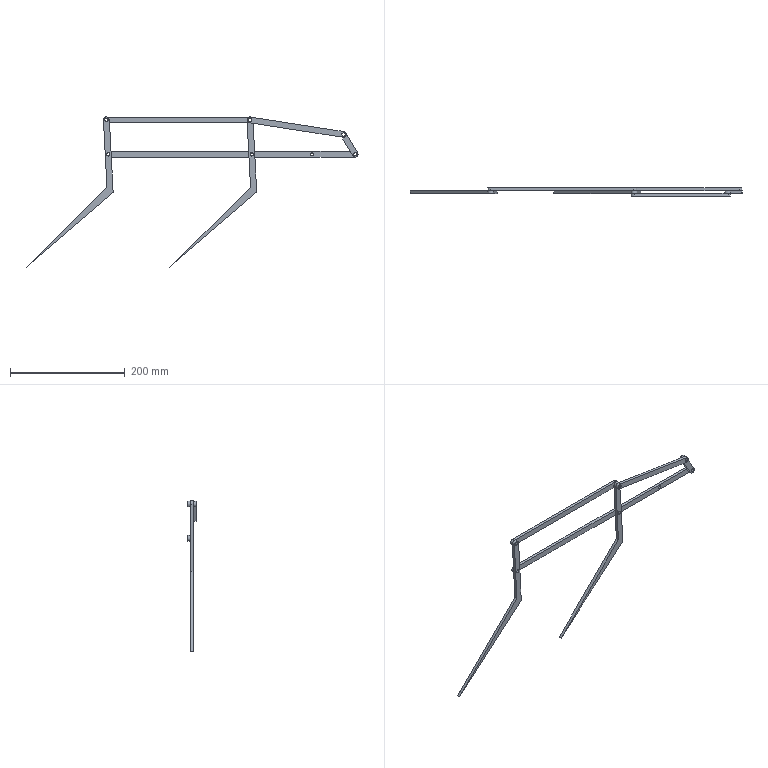Assembly | NX | mm | 6 component files | 6 solids | 52 faces | box 578.16 x 15 x 261.36 mm | volume 70457 mm3 | plane 28 | cylinder 24 | commonest cylinder face diameters 5.929 x12 10 x8 10.285 x2 5 x2
Bill of materials:
unnamed part 1 | 1 |  | Short, thick flat link plate with rounded ends and two through-holes, one at each end
unnamed part 2 | 1 |  | Long, slender flat bar with rounded ends and four small through-holes along its length
unnamed part 3 | 2 |  | Thin flat bent bar with two straight segments at an obtuse angle. One arm has a rounded end with two holes; the other arm tapers to a sharp point
unnamed part 4 | 1 |  | Long flat link bar with rounded ends and one through-hole at each end
unnamed part 5 | 1 |  | Long, slender flat bar with rounded ends and one through-hole at each end
Mates:
1. fix | 1 1 component
2. distance | 60 2 face | 1 1 face
3. touch align | 60 2 face | 1 1 face
4. touch align | 250 1 face | 60 2 face
5. touch align | 165 1 face | 40 1 face
6. touch align | 165 1 face | 60 2 face
7. distance | 165 1 face | 60 2 face
8. touch align | 60 1 face | 1 1 face
9. touch align | 40 1 face | 1 1 face
10. touch align | 1 1 face | 40 1 face
11. distance | 60 1 face | 1 1 face
12. distance | 250 1 face | 60 2 face
13. touch align | 250 1 face | 60 1 face